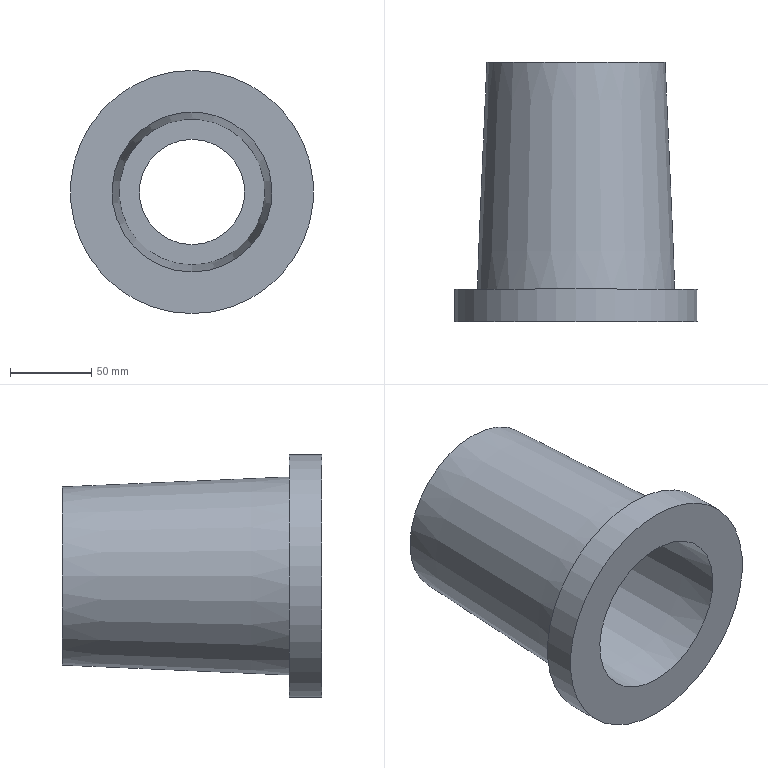Component | NX | BASE | 1 solid | 17 faces | box 150 x 160 x 150 mm | volume 897725 mm3 | cylinder 6 | cone 6 | plane 5 | commonest cylinder face diameters 82 x2 8.5 x2 150 x1 65 x1
STEP:
#1=CARTESIAN_POINT('',(0.,0.,0.));
#2=DIRECTION('',(0.,0.,1.));
#3=DIRECTION('',(1.,0.,0.));
#4=AXIS2_PLACEMENT_3D('',#1,#2,#3);
#5=CARTESIAN_POINT('',(-4.244,159.25,-40.78));
#6=VERTEX_POINT('',#5);
#7=CARTESIAN_POINT('',(-4.991,160.,-40.695));
#8=VERTEX_POINT('',#7);
#9=CARTESIAN_POINT('',(-4.244,159.25,-40.78));
#10=CARTESIAN_POINT('',(-4.493,159.5,-40.754));
#11=CARTESIAN_POINT('',(-4.742,159.75,-40.726));
#12=CARTESIAN_POINT('',(-4.991,160.,-40.695));
#13=B_SPLINE_CURVE_WITH_KNOTS('',3,(#9,#10,#11,#12),.UNSPECIFIED.,.F.,.F.,(4,4),(0.,1.),.PIECEWISE_BEZIER_KNOTS.);
#14=CARTESIAN_POINT('',(0.,0.,0.));
#15=DIRECTION('',(0.,-1.,0.));
#16=DIRECTION('',(0.,0.,-1.));
#17=AXIS2_PLACEMENT_3D('',#14,#15,#16);
#18=CYLINDRICAL_SURFACE('',#17,41.);
#19=CARTESIAN_POINT('',(6.179,-159.25));
#20=CARTESIAN_POINT('',(6.161,-160.));
#21=B_SPLINE_CURVE_WITH_KNOTS('',1,(#19,#20),.UNSPECIFIED.,.F.,.F.,(2,2),(0.,1.),.PIECEWISE_BEZIER_KNOTS.);
#22=(GEOMETRIC_REPRESENTATION_CONTEXT(2)PARAMETRIC_REPRESENTATION_CONTEXT()REPRESENTATION_CONTEXT('',''));
#23=DEFINITIONAL_REPRESENTATION('',(#21),#22);
#24=PCURVE('',#18,#23);
#25=CARTESIAN_POINT('',(0.,160.,-41.));
#26=DIRECTION('',(0.,1.,0.));
#27=DIRECTION('',(0.,0.,1.));
#28=AXIS2_PLACEMENT_3D('',#25,#26,#27);
#29=CONICAL_SURFACE('',#28,5.,0.7854);
#30=CARTESIAN_POINT('',(4.764,-0.75));
#31=CARTESIAN_POINT('',(4.773,0.));
#32=B_SPLINE_CURVE_WITH_KNOTS('',1,(#30,#31),.UNSPECIFIED.,.F.,.F.,(2,2),(0.,1.),.PIECEWISE_BEZIER_KNOTS.);
#33=(GEOMETRIC_REPRESENTATION_CONTEXT(2)PARAMETRIC_REPRESENTATION_CONTEXT()REPRESENTATION_CONTEXT('',''));
#34=DEFINITIONAL_REPRESENTATION('',(#32),#33);
#35=PCURVE('',#29,#34);
#36=SURFACE_CURVE('',#13,(#24,#35),.PCURVE_S1.);
#37=EDGE_CURVE('',#6,#8,#36,.T.);
#38=ORIENTED_EDGE('',*,*,#37,.F.);
#39=CARTESIAN_POINT('',(-4.244,140.,-40.78));
#40=VERTEX_POINT('',#39);
#41=CARTESIAN_POINT('',(-4.244,150.,-40.78));
#42=DIRECTION('',(0.,1.,0.));
#43=VECTOR('',#42,1.);
#44=LINE('',#41,#43);
#45=CARTESIAN_POINT('',(6.179,-150.));
#46=DIRECTION('',(0.,-1.));
#47=VECTOR('',#46,1.);
#48=LINE('',#45,#47);
#49=(GEOMETRIC_REPRESENTATION_CONTEXT(2)PARAMETRIC_REPRESENTATION_CONTEXT()REPRESENTATION_CONTEXT('',''));
#50=DEFINITIONAL_REPRESENTATION('',(#48),#49);
#51=PCURVE('',#18,#50);
#52=CARTESIAN_POINT('',(0.,160.,-41.));
#53=DIRECTION('',(0.,-1.,0.));
#54=DIRECTION('',(0.,0.,-1.));
#55=AXIS2_PLACEMENT_3D('',#52,#53,#54);
#56=CYLINDRICAL_SURFACE('',#55,4.25);
#57=CARTESIAN_POINT('',(-1.623,10.));
#58=DIRECTION('',(0.,-1.));
#59=VECTOR('',#58,1.);
#60=LINE('',#57,#59);
#61=(GEOMETRIC_REPRESENTATION_CONTEXT(2)PARAMETRIC_REPRESENTATION_CONTEXT()REPRESENTATION_CONTEXT('',''));
#62=DEFINITIONAL_REPRESENTATION('',(#60),#61);
#63=PCURVE('',#56,#62);
#64=SURFACE_CURVE('',#44,(#51,#63),.PCURVE_S1.);
#65=EDGE_CURVE('',#40,#6,#64,.T.);
#66=ORIENTED_EDGE('',*,*,#65,.F.);
#67=CARTESIAN_POINT('',(-4.244,140.,40.78));
#68=VERTEX_POINT('',#67);
#69=CARTESIAN_POINT('',(0.,140.,0.));
#70=DIRECTION('',(0.,-1.,0.));
#71=DIRECTION('',(0.,0.,-1.));
#72=AXIS2_PLACEMENT_3D('',#69,#70,#71);
#73=CIRCLE('',#72,41.);
#74=CARTESIAN_POINT('',(-0.,-140.));
#75=DIRECTION('',(1.,0.));
#76=VECTOR('',#75,1.);
#77=LINE('',#74,#76);
#78=(GEOMETRIC_REPRESENTATION_CONTEXT(2)PARAMETRIC_REPRESENTATION_CONTEXT()REPRESENTATION_CONTEXT('',''));
#79=DEFINITIONAL_REPRESENTATION('',(#77),#78);
#80=PCURVE('',#18,#79);
#81=CARTESIAN_POINT('',(-32.5,140.,0.));
#82=DIRECTION('',(0.,-1.,0.));
#83=DIRECTION('',(0.,0.,-1.));
#84=AXIS2_PLACEMENT_3D('',#81,#82,#83);
#85=PLANE('',#84);
#86=CARTESIAN_POINT('',(0.,32.5));
#87=DIRECTION('',(1.,0.));
#88=AXIS2_PLACEMENT_2D('',#86,#87);
#89=CIRCLE('',#88,41.);
#90=(GEOMETRIC_REPRESENTATION_CONTEXT(2)PARAMETRIC_REPRESENTATION_CONTEXT()REPRESENTATION_CONTEXT('',''));
#91=DEFINITIONAL_REPRESENTATION('',(#89),#90);
#92=PCURVE('',#85,#91);
#93=SURFACE_CURVE('',#73,(#80,#92),.PCURVE_S1.);
#94=EDGE_CURVE('',#68,#40,#93,.T.);
#95=ORIENTED_EDGE('',*,*,#94,.F.);
#96=CARTESIAN_POINT('',(-4.244,159.25,40.78));
#97=VERTEX_POINT('',#96);
#98=CARTESIAN_POINT('',(-4.244,150.,40.78));
#99=DIRECTION('',(0.,-1.,0.));
#100=VECTOR('',#99,1.);
#101=LINE('',#98,#100);
#102=CARTESIAN_POINT('',(3.245,-150.));
#103=DIRECTION('',(0.,1.));
#104=VECTOR('',#103,1.);
#105=LINE('',#102,#104);
#106=(GEOMETRIC_REPRESENTATION_CONTEXT(2)PARAMETRIC_REPRESENTATION_CONTEXT()REPRESENTATION_CONTEXT('',''));
#107=DEFINITIONAL_REPRESENTATION('',(#105),#106);
#108=PCURVE('',#18,#107);
#109=CARTESIAN_POINT('',(0.,160.,41.));
#110=DIRECTION('',(0.,-1.,0.));
#111=DIRECTION('',(0.,0.,-1.));
#112=AXIS2_PLACEMENT_3D('',#109,#110,#111);
#113=CYLINDRICAL_SURFACE('',#112,4.25);
#114=CARTESIAN_POINT('',(4.764,10.));
#115=DIRECTION('',(0.,1.));
#116=VECTOR('',#115,1.);
#117=LINE('',#114,#116);
#118=(GEOMETRIC_REPRESENTATION_CONTEXT(2)PARAMETRIC_REPRESENTATION_CONTEXT()REPRESENTATION_CONTEXT('',''));
#119=DEFINITIONAL_REPRESENTATION('',(#117),#118);
#120=PCURVE('',#113,#119);
#121=SURFACE_CURVE('',#101,(#108,#120),.PCURVE_S1.);
#122=EDGE_CURVE('',#97,#68,#121,.T.);
#123=ORIENTED_EDGE('',*,*,#122,.F.);
#124=CARTESIAN_POINT('',(-4.991,160.,40.695));
#125=VERTEX_POINT('',#124);
#126=CARTESIAN_POINT('',(-4.991,160.,40.695));
#127=CARTESIAN_POINT('',(-4.742,159.75,40.726));
#128=CARTESIAN_POINT('',(-4.493,159.5,40.754));
#129=CARTESIAN_POINT('',(-4.244,159.25,40.78));
#130=B_SPLINE_CURVE_WITH_KNOTS('',3,(#126,#127,#128,#129),.UNSPECIFIED.,.F.,.F.,(4,4),(0.,1.),.PIECEWISE_BEZIER_KNOTS.);
#131=CARTESIAN_POINT('',(3.264,-160.));
#132=CARTESIAN_POINT('',(3.245,-159.25));
#133=B_SPLINE_CURVE_WITH_KNOTS('',1,(#131,#132),.UNSPECIFIED.,.F.,.F.,(2,2),(0.,1.),.PIECEWISE_BEZIER_KNOTS.);
#134=(GEOMETRIC_REPRESENTATION_CONTEXT(2)PARAMETRIC_REPRESENTATION_CONTEXT()REPRESENTATION_CONTEXT('',''));
#135=DEFINITIONAL_REPRESENTATION('',(#133),#134);
#136=PCURVE('',#18,#135);
#137=CARTESIAN_POINT('',(0.,160.,41.));
#138=DIRECTION('',(0.,1.,0.));
#139=DIRECTION('',(0.,0.,1.));
#140=AXIS2_PLACEMENT_3D('',#137,#138,#139);
#141=CONICAL_SURFACE('',#140,5.,0.7854);
#142=CARTESIAN_POINT('',(-1.632,0.));
#143=CARTESIAN_POINT('',(-1.623,-0.75));
#144=B_SPLINE_CURVE_WITH_KNOTS('',1,(#142,#143),.UNSPECIFIED.,.F.,.F.,(2,2),(0.,1.),.PIECEWISE_BEZIER_KNOTS.);
#145=(GEOMETRIC_REPRESENTATION_CONTEXT(2)PARAMETRIC_REPRESENTATION_CONTEXT()REPRESENTATION_CONTEXT('',''));
#146=DEFINITIONAL_REPRESENTATION('',(#144),#145);
#147=PCURVE('',#141,#146);
#148=SURFACE_CURVE('',#130,(#136,#147),.PCURVE_S1.);
#149=EDGE_CURVE('',#125,#97,#148,.T.);
#150=ORIENTED_EDGE('',*,*,#149,.F.);
#151=CARTESIAN_POINT('',(0.,160.,0.));
#152=DIRECTION('',(0.,-1.,0.));
#153=DIRECTION('',(0.,0.,-1.));
#154=AXIS2_PLACEMENT_3D('',#151,#152,#153);
#155=CIRCLE('',#154,41.);
#156=CARTESIAN_POINT('',(-0.,-160.));
#157=DIRECTION('',(1.,0.));
#158=VECTOR('',#157,1.);
#159=LINE('',#156,#158);
#160=(GEOMETRIC_REPRESENTATION_CONTEXT(2)PARAMETRIC_REPRESENTATION_CONTEXT()REPRESENTATION_CONTEXT('',''));
#161=DEFINITIONAL_REPRESENTATION('',(#159),#160);
#162=PCURVE('',#18,#161);
#163=CARTESIAN_POINT('',(-41.,160.,0.));
#164=DIRECTION('',(0.,-1.,0.));
#165=DIRECTION('',(0.,0.,-1.));
#166=AXIS2_PLACEMENT_3D('',#163,#164,#165);
#167=PLANE('',#166);
#168=CARTESIAN_POINT('',(0.,41.));
#169=DIRECTION('',(1.,0.));
#170=AXIS2_PLACEMENT_2D('',#168,#169);
#171=CIRCLE('',#170,41.);
#172=(GEOMETRIC_REPRESENTATION_CONTEXT(2)PARAMETRIC_REPRESENTATION_CONTEXT()REPRESENTATION_CONTEXT('',''));
#173=DEFINITIONAL_REPRESENTATION('',(#171),#172);
#174=PCURVE('',#167,#173);
#175=SURFACE_CURVE('',#155,(#162,#174),.PCURVE_S1.);
#176=EDGE_CURVE('',#125,#8,#175,.T.);
#177=ORIENTED_EDGE('',*,*,#176,.T.);
#178=EDGE_LOOP('',(#38,#66,#95,#123,#150,#177));
#179=FACE_BOUND('',#178,.F.);
#180=ADVANCED_FACE('',(#179),#18,.F.);
#181=CARTESIAN_POINT('',(0.,20.,-61.113));
#182=VERTEX_POINT('',#181);
#183=CARTESIAN_POINT('',(0.,20.,0.));
#184=DIRECTION('',(0.,-1.,0.));
#185=DIRECTION('',(0.,0.,-1.));
#186=AXIS2_PLACEMENT_3D('',#183,#184,#185);
#187=CIRCLE('',#186,61.113);
#188=CARTESIAN_POINT('',(0.,160.,0.));
#189=DIRECTION('',(0.,-1.,0.));
#190=DIRECTION('',(0.,0.,-1.));
#191=AXIS2_PLACEMENT_3D('',#188,#189,#190);
#192=CONICAL_SURFACE('',#191,55.,0.04363);
#193=CARTESIAN_POINT('',(0.,140.));
#194=DIRECTION('',(1.,0.));
#195=VECTOR('',#194,1.);
#196=LINE('',#193,#195);
#197=(GEOMETRIC_REPRESENTATION_CONTEXT(2)PARAMETRIC_REPRESENTATION_CONTEXT()REPRESENTATION_CONTEXT('',''));
#198=DEFINITIONAL_REPRESENTATION('',(#196),#197);
#199=PCURVE('',#192,#198);
#200=CARTESIAN_POINT('',(-61.113,20.,0.));
#201=DIRECTION('',(0.,-1.,0.));
#202=DIRECTION('',(0.,0.,-1.));
#203=AXIS2_PLACEMENT_3D('',#200,#201,#202);
#204=PLANE('',#203);
#205=CARTESIAN_POINT('',(0.,61.113));
#206=DIRECTION('',(1.,0.));
#207=AXIS2_PLACEMENT_2D('',#205,#206);
#208=CIRCLE('',#207,61.113);
#209=(GEOMETRIC_REPRESENTATION_CONTEXT(2)PARAMETRIC_REPRESENTATION_CONTEXT()REPRESENTATION_CONTEXT('',''));
#210=DEFINITIONAL_REPRESENTATION('',(#208),#209);
#211=PCURVE('',#204,#210);
#212=SURFACE_CURVE('',#187,(#199,#211),.PCURVE_S1.);
#213=EDGE_CURVE('',#182,#182,#212,.T.);
#214=ORIENTED_EDGE('',*,*,#213,.F.);
#215=CARTESIAN_POINT('',(0.,160.,-55.));
#216=VERTEX_POINT('',#215);
#217=CARTESIAN_POINT('',(-0.,160.,-55.));
#218=CARTESIAN_POINT('',(-0.,20.,-61.113));
#219=B_SPLINE_CURVE_WITH_KNOTS('',1,(#217,#218),.UNSPECIFIED.,.F.,.F.,(2,2),(0.,140.133),.PIECEWISE_BEZIER_KNOTS.);
#220=CARTESIAN_POINT('',(0.,0.));
#221=DIRECTION('',(0.,1.));
#222=VECTOR('',#221,1.);
#223=LINE('',#220,#222);
#224=(GEOMETRIC_REPRESENTATION_CONTEXT(2)PARAMETRIC_REPRESENTATION_CONTEXT()REPRESENTATION_CONTEXT('',''));
#225=DEFINITIONAL_REPRESENTATION('',(#223),#224);
#226=PCURVE('',#192,#225);
#227=CARTESIAN_POINT('',(6.283,0.));
#228=DIRECTION('',(0.,1.));
#229=VECTOR('',#228,1.);
#230=LINE('',#227,#229);
#231=(GEOMETRIC_REPRESENTATION_CONTEXT(2)PARAMETRIC_REPRESENTATION_CONTEXT()REPRESENTATION_CONTEXT('',''));
#232=DEFINITIONAL_REPRESENTATION('',(#230),#231);
#233=PCURVE('',#192,#232);
#234=SEAM_CURVE('',#219,(#226,#233),.PCURVE_S1.);
#235=EDGE_CURVE('',#216,#182,#234,.T.);
#236=ORIENTED_EDGE('',*,*,#235,.F.);
#237=CARTESIAN_POINT('',(0.,160.,0.));
#238=DIRECTION('',(0.,-1.,0.));
#239=DIRECTION('',(0.,0.,-1.));
#240=AXIS2_PLACEMENT_3D('',#237,#238,#239);
#241=CIRCLE('',#240,55.);
#242=CARTESIAN_POINT('',(0.,0.));
#243=DIRECTION('',(1.,0.));
#244=VECTOR('',#243,1.);
#245=LINE('',#242,#244);
#246=(GEOMETRIC_REPRESENTATION_CONTEXT(2)PARAMETRIC_REPRESENTATION_CONTEXT()REPRESENTATION_CONTEXT('',''));
#247=DEFINITIONAL_REPRESENTATION('',(#245),#246);
#248=PCURVE('',#192,#247);
#249=CARTESIAN_POINT('',(0.,41.));
#250=DIRECTION('',(1.,0.));
#251=AXIS2_PLACEMENT_2D('',#249,#250);
#252=CIRCLE('',#251,55.);
#253=(GEOMETRIC_REPRESENTATION_CONTEXT(2)PARAMETRIC_REPRESENTATION_CONTEXT()REPRESENTATION_CONTEXT('',''));
#254=DEFINITIONAL_REPRESENTATION('',(#252),#253);
#255=PCURVE('',#167,#254);
#256=SURFACE_CURVE('',#241,(#248,#255),.PCURVE_S1.);
#257=EDGE_CURVE('',#216,#216,#256,.T.);
#258=ORIENTED_EDGE('',*,*,#257,.T.);
#259=ORIENTED_EDGE('',*,*,#235,.T.);
#260=EDGE_LOOP('',(#214,#236,#258,#259));
#261=FACE_BOUND('',#260,.T.);
#262=ADVANCED_FACE('',(#261),#192,.T.);
#263=CARTESIAN_POINT('',(0.,20.,-75.));
#264=VERTEX_POINT('',#263);
#265=CARTESIAN_POINT('',(0.,20.,0.));
#266=DIRECTION('',(0.,-1.,0.));
#267=DIRECTION('',(0.,0.,-1.));
#268=AXIS2_PLACEMENT_3D('',#265,#266,#267);
#269=CIRCLE('',#268,75.);
#270=CARTESIAN_POINT('',(0.,61.113));
#271=DIRECTION('',(1.,0.));
#272=AXIS2_PLACEMENT_2D('',#270,#271);
#273=CIRCLE('',#272,75.);
#274=(GEOMETRIC_REPRESENTATION_CONTEXT(2)PARAMETRIC_REPRESENTATION_CONTEXT()REPRESENTATION_CONTEXT('',''));
#275=DEFINITIONAL_REPRESENTATION('',(#273),#274);
#276=PCURVE('',#204,#275);
#277=CARTESIAN_POINT('',(0.,0.,0.));
#278=DIRECTION('',(0.,-1.,0.));
#279=DIRECTION('',(0.,0.,-1.));
#280=AXIS2_PLACEMENT_3D('',#277,#278,#279);
#281=CYLINDRICAL_SURFACE('',#280,75.);
#282=CARTESIAN_POINT('',(0.,-20.));
#283=DIRECTION('',(1.,0.));
#284=VECTOR('',#283,1.);
#285=LINE('',#282,#284);
#286=(GEOMETRIC_REPRESENTATION_CONTEXT(2)PARAMETRIC_REPRESENTATION_CONTEXT()REPRESENTATION_CONTEXT('',''));
#287=DEFINITIONAL_REPRESENTATION('',(#285),#286);
#288=PCURVE('',#281,#287);
#289=SURFACE_CURVE('',#269,(#276,#288),.PCURVE_S1.);
#290=EDGE_CURVE('',#264,#264,#289,.T.);
#291=ORIENTED_EDGE('',*,*,#290,.F.);
#292=EDGE_LOOP('',(#291));
#293=FACE_BOUND('',#292,.T.);
#294=ORIENTED_EDGE('',*,*,#213,.T.);
#295=EDGE_LOOP('',(#294));
#296=FACE_BOUND('',#295,.T.);
#297=ADVANCED_FACE('',(#293,#296),#204,.F.);
#298=CARTESIAN_POINT('',(0.,-0.,-75.));
#299=VERTEX_POINT('',#298);
#300=CARTESIAN_POINT('',(0.,-0.,0.));
#301=DIRECTION('',(0.,-1.,0.));
#302=DIRECTION('',(0.,0.,-1.));
#303=AXIS2_PLACEMENT_3D('',#300,#301,#302);
#304=CIRCLE('',#303,75.);
#305=CARTESIAN_POINT('',(0.,0.));
#306=DIRECTION('',(1.,0.));
#307=VECTOR('',#306,1.);
#308=LINE('',#305,#307);
#309=(GEOMETRIC_REPRESENTATION_CONTEXT(2)PARAMETRIC_REPRESENTATION_CONTEXT()REPRESENTATION_CONTEXT('',''));
#310=DEFINITIONAL_REPRESENTATION('',(#308),#309);
#311=PCURVE('',#281,#310);
#312=CARTESIAN_POINT('',(-75.,-0.,0.));
#313=DIRECTION('',(0.,1.,0.));
#314=DIRECTION('',(0.,0.,1.));
#315=AXIS2_PLACEMENT_3D('',#312,#313,#314);
#316=PLANE('',#315);
#317=CARTESIAN_POINT('',(-75.,75.));
#318=CARTESIAN_POINT('',(-75.,204.904));
#319=CARTESIAN_POINT('',(37.5,139.952));
#320=CARTESIAN_POINT('',(150.,75.));
#321=CARTESIAN_POINT('',(37.5,10.048));
#322=CARTESIAN_POINT('',(-75.,-54.904));
#323=CARTESIAN_POINT('',(-75.,75.));
#324=(BOUNDED_CURVE()B_SPLINE_CURVE(2,(#317,#318,#319,#320,#321,#322,#323),.UNSPECIFIED.,.T.,.F.)B_SPLINE_CURVE_WITH_KNOTS((1,2,2,2,2,1),(-2.094,0.,2.094,4.189,6.283,8.378),.UNSPECIFIED.)CURVE()GEOMETRIC_REPRESENTATION_ITEM()RATIONAL_B_SPLINE_CURVE((1.,0.5,1.,0.5,1.,0.5,1.))REPRESENTATION_ITEM(''));
#325=(GEOMETRIC_REPRESENTATION_CONTEXT(2)PARAMETRIC_REPRESENTATION_CONTEXT()REPRESENTATION_CONTEXT('',''));
#326=DEFINITIONAL_REPRESENTATION('',(#324),#325);
#327=PCURVE('',#316,#326);
#328=SURFACE_CURVE('',#304,(#311,#327),.PCURVE_S1.);
#329=EDGE_CURVE('',#299,#299,#328,.T.);
#330=ORIENTED_EDGE('',*,*,#329,.F.);
#331=CARTESIAN_POINT('',(-0.,20.,-75.));
#332=CARTESIAN_POINT('',(-0.,-0.,-75.));
#333=B_SPLINE_CURVE_WITH_KNOTS('',1,(#331,#332),.UNSPECIFIED.,.F.,.F.,(2,2),(-20.,0.),.PIECEWISE_BEZIER_KNOTS.);
#334=CARTESIAN_POINT('',(0.,0.));
#335=DIRECTION('',(0.,1.));
#336=VECTOR('',#335,1.);
#337=LINE('',#334,#336);
#338=(GEOMETRIC_REPRESENTATION_CONTEXT(2)PARAMETRIC_REPRESENTATION_CONTEXT()REPRESENTATION_CONTEXT('',''));
#339=DEFINITIONAL_REPRESENTATION('',(#337),#338);
#340=PCURVE('',#281,#339);
#341=CARTESIAN_POINT('',(6.283,0.));
#342=DIRECTION('',(0.,1.));
#343=VECTOR('',#342,1.);
#344=LINE('',#341,#343);
#345=(GEOMETRIC_REPRESENTATION_CONTEXT(2)PARAMETRIC_REPRESENTATION_CONTEXT()REPRESENTATION_CONTEXT('',''));
#346=DEFINITIONAL_REPRESENTATION('',(#344),#345);
#347=PCURVE('',#281,#346);
#348=SEAM_CURVE('',#333,(#340,#347),.PCURVE_S1.);
#349=EDGE_CURVE('',#264,#299,#348,.T.);
#350=ORIENTED_EDGE('',*,*,#349,.F.);
#351=ORIENTED_EDGE('',*,*,#290,.T.);
#352=ORIENTED_EDGE('',*,*,#349,.T.);
#353=EDGE_LOOP('',(#330,#350,#351,#352));
#354=FACE_BOUND('',#353,.T.);
#355=ADVANCED_FACE('',(#354),#281,.T.);
#356=CARTESIAN_POINT('',(0.,-0.,-49.366));
#357=VERTEX_POINT('',#356);
#358=CARTESIAN_POINT('',(0.,-0.,0.));
#359=DIRECTION('',(0.,-1.,0.));
#360=DIRECTION('',(0.,0.,-1.));
#361=AXIS2_PLACEMENT_3D('',#358,#359,#360);
#362=CIRCLE('',#361,49.366);
#363=CARTESIAN_POINT('',(-49.366,75.));
#364=CARTESIAN_POINT('',(-49.366,160.505));
#365=CARTESIAN_POINT('',(24.683,117.752));
#366=CARTESIAN_POINT('',(98.732,75.));
#367=CARTESIAN_POINT('',(24.683,32.248));
#368=CARTESIAN_POINT('',(-49.366,-10.505));
#369=CARTESIAN_POINT('',(-49.366,75.));
#370=(BOUNDED_CURVE()B_SPLINE_CURVE(2,(#363,#364,#365,#366,#367,#368,#369),.UNSPECIFIED.,.T.,.F.)B_SPLINE_CURVE_WITH_KNOTS((1,2,2,2,2,1),(-2.094,0.,2.094,4.189,6.283,8.378),.UNSPECIFIED.)CURVE()GEOMETRIC_REPRESENTATION_ITEM()RATIONAL_B_SPLINE_CURVE((1.,0.5,1.,0.5,1.,0.5,1.))REPRESENTATION_ITEM(''));
#371=(GEOMETRIC_REPRESENTATION_CONTEXT(2)PARAMETRIC_REPRESENTATION_CONTEXT()REPRESENTATION_CONTEXT('',''));
#372=DEFINITIONAL_REPRESENTATION('',(#370),#371);
#373=PCURVE('',#316,#372);
#374=CARTESIAN_POINT('',(0.,-0.,0.));
#375=DIRECTION('',(0.,-1.,0.));
#376=DIRECTION('',(0.,0.,-1.));
#377=AXIS2_PLACEMENT_3D('',#374,#375,#376);
#378=CONICAL_SURFACE('',#377,49.366,0.04363);
#379=CARTESIAN_POINT('',(0.,0.));
#380=DIRECTION('',(1.,0.));
#381=VECTOR('',#380,1.);
#382=LINE('',#379,#381);
#383=(GEOMETRIC_REPRESENTATION_CONTEXT(2)PARAMETRIC_REPRESENTATION_CONTEXT()REPRESENTATION_CONTEXT('',''));
#384=DEFINITIONAL_REPRESENTATION('',(#382),#383);
#385=PCURVE('',#378,#384);
#386=SURFACE_CURVE('',#362,(#373,#385),.PCURVE_S1.);
#387=EDGE_CURVE('',#357,#357,#386,.T.);
#388=ORIENTED_EDGE('',*,*,#387,.F.);
#389=EDGE_LOOP('',(#388));
#390=FACE_BOUND('',#389,.T.);
#391=ORIENTED_EDGE('',*,*,#329,.T.);
#392=EDGE_LOOP('',(#391));
#393=FACE_BOUND('',#392,.T.);
#394=ADVANCED_FACE('',(#390,#393),#316,.F.);
#395=CARTESIAN_POINT('',(0.,100.,-45.));
#396=VERTEX_POINT('',#395);
#397=CARTESIAN_POINT('',(0.,100.,0.));
#398=DIRECTION('',(0.,-1.,0.));
#399=DIRECTION('',(0.,0.,-1.));
#400=AXIS2_PLACEMENT_3D('',#397,#398,#399);
#401=CIRCLE('',#400,45.);
#402=CARTESIAN_POINT('',(0.,-100.));
#403=DIRECTION('',(1.,0.));
#404=VECTOR('',#403,1.);
#405=LINE('',#402,#404);
#406=(GEOMETRIC_REPRESENTATION_CONTEXT(2)PARAMETRIC_REPRESENTATION_CONTEXT()REPRESENTATION_CONTEXT('',''));
#407=DEFINITIONAL_REPRESENTATION('',(#405),#406);
#408=PCURVE('',#378,#407);
#409=CARTESIAN_POINT('',(-45.,100.,0.));
#410=DIRECTION('',(0.,1.,0.));
#411=DIRECTION('',(0.,0.,1.));
#412=AXIS2_PLACEMENT_3D('',#409,#410,#411);
#413=PLANE('',#412);
#414=CARTESIAN_POINT('',(-45.,45.));
#415=CARTESIAN_POINT('',(-45.,122.942));
#416=CARTESIAN_POINT('',(22.5,83.971));
#417=CARTESIAN_POINT('',(90.,45.));
#418=CARTESIAN_POINT('',(22.5,6.029));
#419=CARTESIAN_POINT('',(-45.,-32.942));
#420=CARTESIAN_POINT('',(-45.,45.));
#421=(BOUNDED_CURVE()B_SPLINE_CURVE(2,(#414,#415,#416,#417,#418,#419,#420),.UNSPECIFIED.,.T.,.F.)B_SPLINE_CURVE_WITH_KNOTS((1,2,2,2,2,1),(-2.094,0.,2.094,4.189,6.283,8.378),.UNSPECIFIED.)CURVE()GEOMETRIC_REPRESENTATION_ITEM()RATIONAL_B_SPLINE_CURVE((1.,0.5,1.,0.5,1.,0.5,1.))REPRESENTATION_ITEM(''));
#422=(GEOMETRIC_REPRESENTATION_CONTEXT(2)PARAMETRIC_REPRESENTATION_CONTEXT()REPRESENTATION_CONTEXT('',''));
#423=DEFINITIONAL_REPRESENTATION('',(#421),#422);
#424=PCURVE('',#413,#423);
#425=SURFACE_CURVE('',#401,(#408,#424),.PCURVE_S1.);
#426=EDGE_CURVE('',#396,#396,#425,.T.);
#427=ORIENTED_EDGE('',*,*,#426,.T.);
#428=CARTESIAN_POINT('',(0.,100.,-45.));
#429=CARTESIAN_POINT('',(0.,-0.,-49.366));
#430=B_SPLINE_CURVE_WITH_KNOTS('',1,(#428,#429),.UNSPECIFIED.,.F.,.F.,(2,2),(-100.095,0.),.PIECEWISE_BEZIER_KNOTS.);
#431=CARTESIAN_POINT('',(6.283,0.));
#432=DIRECTION('',(0.,1.));
#433=VECTOR('',#432,1.);
#434=LINE('',#431,#433);
#435=(GEOMETRIC_REPRESENTATION_CONTEXT(2)PARAMETRIC_REPRESENTATION_CONTEXT()REPRESENTATION_CONTEXT('',''));
#436=DEFINITIONAL_REPRESENTATION('',(#434),#435);
#437=PCURVE('',#378,#436);
#438=CARTESIAN_POINT('',(0.,0.));
#439=DIRECTION('',(0.,1.));
#440=VECTOR('',#439,1.);
#441=LINE('',#438,#440);
#442=(GEOMETRIC_REPRESENTATION_CONTEXT(2)PARAMETRIC_REPRESENTATION_CONTEXT()REPRESENTATION_CONTEXT('',''));
#443=DEFINITIONAL_REPRESENTATION('',(#441),#442);
#444=PCURVE('',#378,#443);
#445=SEAM_CURVE('',#430,(#437,#444),.PCURVE_S1.);
#446=EDGE_CURVE('',#396,#357,#445,.T.);
#447=ORIENTED_EDGE('',*,*,#446,.T.);
#448=ORIENTED_EDGE('',*,*,#387,.F.);
#449=ORIENTED_EDGE('',*,*,#446,.F.);
#450=EDGE_LOOP('',(#427,#447,#448,#449));
#451=FACE_BOUND('',#450,.F.);
#452=ADVANCED_FACE('',(#451),#378,.F.);
#453=CARTESIAN_POINT('',(0.,100.,-32.5));
#454=VERTEX_POINT('',#453);
#455=CARTESIAN_POINT('',(0.,100.,0.));
#456=DIRECTION('',(0.,-1.,0.));
#457=DIRECTION('',(0.,0.,-1.));
#458=AXIS2_PLACEMENT_3D('',#455,#456,#457);
#459=CIRCLE('',#458,32.5);
#460=CARTESIAN_POINT('',(-32.5,45.));
#461=CARTESIAN_POINT('',(-32.5,101.292));
#462=CARTESIAN_POINT('',(16.25,73.146));
#463=CARTESIAN_POINT('',(65.,45.));
#464=CARTESIAN_POINT('',(16.25,16.854));
#465=CARTESIAN_POINT('',(-32.5,-11.292));
#466=CARTESIAN_POINT('',(-32.5,45.));
#467=(BOUNDED_CURVE()B_SPLINE_CURVE(2,(#460,#461,#462,#463,#464,#465,#466),.UNSPECIFIED.,.T.,.F.)B_SPLINE_CURVE_WITH_KNOTS((1,2,2,2,2,1),(-2.094,0.,2.094,4.189,6.283,8.378),.UNSPECIFIED.)CURVE()GEOMETRIC_REPRESENTATION_ITEM()RATIONAL_B_SPLINE_CURVE((1.,0.5,1.,0.5,1.,0.5,1.))REPRESENTATION_ITEM(''));
#468=(GEOMETRIC_REPRESENTATION_CONTEXT(2)PARAMETRIC_REPRESENTATION_CONTEXT()REPRESENTATION_CONTEXT('',''));
#469=DEFINITIONAL_REPRESENTATION('',(#467),#468);
#470=PCURVE('',#413,#469);
#471=CARTESIAN_POINT('',(0.,0.,0.));
#472=DIRECTION('',(0.,-1.,0.));
#473=DIRECTION('',(0.,0.,-1.));
#474=AXIS2_PLACEMENT_3D('',#471,#472,#473);
#475=CYLINDRICAL_SURFACE('',#474,32.5);
#476=CARTESIAN_POINT('',(0.,-100.));
#477=DIRECTION('',(1.,0.));
#478=VECTOR('',#477,1.);
#479=LINE('',#476,#478);
#480=(GEOMETRIC_REPRESENTATION_CONTEXT(2)PARAMETRIC_REPRESENTATION_CONTEXT()REPRESENTATION_CONTEXT('',''));
#481=DEFINITIONAL_REPRESENTATION('',(#479),#480);
#482=PCURVE('',#475,#481);
#483=SURFACE_CURVE('',#459,(#470,#482),.PCURVE_S1.);
#484=EDGE_CURVE('',#454,#454,#483,.T.);
#485=ORIENTED_EDGE('',*,*,#484,.F.);
#486=EDGE_LOOP('',(#485));
#487=FACE_BOUND('',#486,.T.);
#488=ORIENTED_EDGE('',*,*,#426,.T.);
#489=EDGE_LOOP('',(#488));
#490=FACE_BOUND('',#489,.T.);
#491=ADVANCED_FACE('',(#487,#490),#413,.F.);
#492=CARTESIAN_POINT('',(0.,140.,-32.5));
#493=VERTEX_POINT('',#492);
#494=CARTESIAN_POINT('',(0.,140.,0.));
#495=DIRECTION('',(0.,-1.,0.));
#496=DIRECTION('',(0.,0.,-1.));
#497=AXIS2_PLACEMENT_3D('',#494,#495,#496);
#498=CIRCLE('',#497,32.5);
#499=CARTESIAN_POINT('',(0.,-140.));
#500=DIRECTION('',(1.,0.));
#501=VECTOR('',#500,1.);
#502=LINE('',#499,#501);
#503=(GEOMETRIC_REPRESENTATION_CONTEXT(2)PARAMETRIC_REPRESENTATION_CONTEXT()REPRESENTATION_CONTEXT('',''));
#504=DEFINITIONAL_REPRESENTATION('',(#502),#503);
#505=PCURVE('',#475,#504);
#506=CARTESIAN_POINT('',(0.,32.5));
#507=DIRECTION('',(1.,0.));
#508=AXIS2_PLACEMENT_2D('',#506,#507);
#509=CIRCLE('',#508,32.5);
#510=(GEOMETRIC_REPRESENTATION_CONTEXT(2)PARAMETRIC_REPRESENTATION_CONTEXT()REPRESENTATION_CONTEXT('',''));
#511=DEFINITIONAL_REPRESENTATION('',(#509),#510);
#512=PCURVE('',#85,#511);
#513=SURFACE_CURVE('',#498,(#505,#512),.PCURVE_S1.);
#514=EDGE_CURVE('',#493,#493,#513,.T.);
#515=ORIENTED_EDGE('',*,*,#514,.T.);
#516=CARTESIAN_POINT('',(0.,140.,-32.5));
#517=CARTESIAN_POINT('',(0.,100.,-32.5));
#518=B_SPLINE_CURVE_WITH_KNOTS('',1,(#516,#517),.UNSPECIFIED.,.F.,.F.,(2,2),(-140.,-100.),.PIECEWISE_BEZIER_KNOTS.);
#519=CARTESIAN_POINT('',(6.283,0.));
#520=DIRECTION('',(0.,1.));
#521=VECTOR('',#520,1.);
#522=LINE('',#519,#521);
#523=(GEOMETRIC_REPRESENTATION_CONTEXT(2)PARAMETRIC_REPRESENTATION_CONTEXT()REPRESENTATION_CONTEXT('',''));
#524=DEFINITIONAL_REPRESENTATION('',(#522),#523);
#525=PCURVE('',#475,#524);
#526=CARTESIAN_POINT('',(0.,0.));
#527=DIRECTION('',(0.,1.));
#528=VECTOR('',#527,1.);
#529=LINE('',#526,#528);
#530=(GEOMETRIC_REPRESENTATION_CONTEXT(2)PARAMETRIC_REPRESENTATION_CONTEXT()REPRESENTATION_CONTEXT('',''));
#531=DEFINITIONAL_REPRESENTATION('',(#529),#530);
#532=PCURVE('',#475,#531);
#533=SEAM_CURVE('',#518,(#525,#532),.PCURVE_S1.);
#534=EDGE_CURVE('',#493,#454,#533,.T.);
#535=ORIENTED_EDGE('',*,*,#534,.T.);
#536=ORIENTED_EDGE('',*,*,#484,.F.);
#537=ORIENTED_EDGE('',*,*,#534,.F.);
#538=EDGE_LOOP('',(#515,#535,#536,#537));
#539=FACE_BOUND('',#538,.F.);
#540=ADVANCED_FACE('',(#539),#475,.F.);
#541=ORIENTED_EDGE('',*,*,#94,.F.);
#542=CARTESIAN_POINT('',(4.244,140.,40.78));
#543=VERTEX_POINT('',#542);
#544=CARTESIAN_POINT('',(0.,140.,41.));
#545=DIRECTION('',(0.,-1.,0.));
#546=DIRECTION('',(0.,0.,-1.));
#547=AXIS2_PLACEMENT_3D('',#544,#545,#546);
#548=CIRCLE('',#547,4.25);
#549=CARTESIAN_POINT('',(-41.,32.5));
#550=DIRECTION('',(1.,0.));
#551=AXIS2_PLACEMENT_2D('',#549,#550);
#552=CIRCLE('',#551,4.25);
#553=(GEOMETRIC_REPRESENTATION_CONTEXT(2)PARAMETRIC_REPRESENTATION_CONTEXT()REPRESENTATION_CONTEXT('',''));
#554=DEFINITIONAL_REPRESENTATION('',(#552),#553);
#555=PCURVE('',#85,#554);
#556=CARTESIAN_POINT('',(0.,140.,41.));
#557=DIRECTION('',(0.,1.,0.));
#558=DIRECTION('',(0.,0.,1.));
#559=AXIS2_PLACEMENT_3D('',#556,#557,#558);
#560=CONICAL_SURFACE('',#559,4.25,1.03);
#561=CARTESIAN_POINT('',(9.425,0.));
#562=DIRECTION('',(-1.,0.));
#563=VECTOR('',#562,1.);
#564=LINE('',#561,#563);
#565=(GEOMETRIC_REPRESENTATION_CONTEXT(2)PARAMETRIC_REPRESENTATION_CONTEXT()REPRESENTATION_CONTEXT('',''));
#566=DEFINITIONAL_REPRESENTATION('',(#564),#565);
#567=PCURVE('',#560,#566);
#568=SURFACE_CURVE('',#548,(#555,#567),.PCURVE_S1.);
#569=EDGE_CURVE('',#68,#543,#568,.T.);
#570=ORIENTED_EDGE('',*,*,#569,.T.);
#571=CARTESIAN_POINT('',(4.244,140.,-40.78));
#572=VERTEX_POINT('',#571);
#573=CARTESIAN_POINT('',(0.,140.,0.));
#574=DIRECTION('',(0.,-1.,0.));
#575=DIRECTION('',(0.,0.,-1.));
#576=AXIS2_PLACEMENT_3D('',#573,#574,#575);
#577=CIRCLE('',#576,41.);
#578=CARTESIAN_POINT('',(0.,32.5));
#579=DIRECTION('',(1.,0.));
#580=AXIS2_PLACEMENT_2D('',#578,#579);
#581=CIRCLE('',#580,41.);
#582=(GEOMETRIC_REPRESENTATION_CONTEXT(2)PARAMETRIC_REPRESENTATION_CONTEXT()REPRESENTATION_CONTEXT('',''));
#583=DEFINITIONAL_REPRESENTATION('',(#581),#582);
#584=PCURVE('',#85,#583);
#585=CARTESIAN_POINT('',(0.,0.,0.));
#586=DIRECTION('',(0.,-1.,0.));
#587=DIRECTION('',(0.,0.,-1.));
#588=AXIS2_PLACEMENT_3D('',#585,#586,#587);
#589=CYLINDRICAL_SURFACE('',#588,41.);
#590=CARTESIAN_POINT('',(0.,-140.));
#591=DIRECTION('',(1.,0.));
#592=VECTOR('',#591,1.);
#593=LINE('',#590,#592);
#594=(GEOMETRIC_REPRESENTATION_CONTEXT(2)PARAMETRIC_REPRESENTATION_CONTEXT()REPRESENTATION_CONTEXT('',''));
#595=DEFINITIONAL_REPRESENTATION('',(#593),#594);
#596=PCURVE('',#589,#595);
#597=SURFACE_CURVE('',#577,(#584,#596),.PCURVE_S1.);
#598=EDGE_CURVE('',#572,#543,#597,.T.);
#599=ORIENTED_EDGE('',*,*,#598,.F.);
#600=CARTESIAN_POINT('',(0.,140.,-36.75));
#601=VERTEX_POINT('',#600);
#602=CARTESIAN_POINT('',(0.,140.,-41.));
#603=DIRECTION('',(0.,-1.,0.));
#604=DIRECTION('',(0.,0.,-1.));
#605=AXIS2_PLACEMENT_3D('',#602,#603,#604);
#606=CIRCLE('',#605,4.25);
#607=CARTESIAN_POINT('',(41.,32.5));
#608=DIRECTION('',(1.,0.));
#609=AXIS2_PLACEMENT_2D('',#607,#608);
#610=CIRCLE('',#609,4.25);
#611=(GEOMETRIC_REPRESENTATION_CONTEXT(2)PARAMETRIC_REPRESENTATION_CONTEXT()REPRESENTATION_CONTEXT('',''));
#612=DEFINITIONAL_REPRESENTATION('',(#610),#611);
#613=PCURVE('',#85,#612);
#614=CARTESIAN_POINT('',(0.,140.,-41.));
#615=DIRECTION('',(0.,1.,0.));
#616=DIRECTION('',(0.,0.,1.));
#617=AXIS2_PLACEMENT_3D('',#614,#615,#616);
#618=CONICAL_SURFACE('',#617,4.25,1.03);
#619=CARTESIAN_POINT('',(3.142,0.));
#620=DIRECTION('',(-1.,0.));
#621=VECTOR('',#620,1.);
#622=LINE('',#619,#621);
#623=(GEOMETRIC_REPRESENTATION_CONTEXT(2)PARAMETRIC_REPRESENTATION_CONTEXT()REPRESENTATION_CONTEXT('',''));
#624=DEFINITIONAL_REPRESENTATION('',(#622),#623);
#625=PCURVE('',#618,#624);
#626=SURFACE_CURVE('',#606,(#613,#625),.PCURVE_S1.);
#627=EDGE_CURVE('',#572,#601,#626,.T.);
#628=ORIENTED_EDGE('',*,*,#627,.T.);
#629=CARTESIAN_POINT('',(0.,140.,-41.));
#630=DIRECTION('',(0.,-1.,0.));
#631=DIRECTION('',(0.,0.,-1.));
#632=AXIS2_PLACEMENT_3D('',#629,#630,#631);
#633=CIRCLE('',#632,4.25);
#634=CARTESIAN_POINT('',(41.,32.5));
#635=DIRECTION('',(1.,0.));
#636=AXIS2_PLACEMENT_2D('',#634,#635);
#637=CIRCLE('',#636,4.25);
#638=(GEOMETRIC_REPRESENTATION_CONTEXT(2)PARAMETRIC_REPRESENTATION_CONTEXT()REPRESENTATION_CONTEXT('',''));
#639=DEFINITIONAL_REPRESENTATION('',(#637),#638);
#640=PCURVE('',#85,#639);
#641=CARTESIAN_POINT('',(9.425,0.));
#642=DIRECTION('',(-1.,0.));
#643=VECTOR('',#642,1.);
#644=LINE('',#641,#643);
#645=(GEOMETRIC_REPRESENTATION_CONTEXT(2)PARAMETRIC_REPRESENTATION_CONTEXT()REPRESENTATION_CONTEXT('',''));
#646=DEFINITIONAL_REPRESENTATION('',(#644),#645);
#647=PCURVE('',#618,#646);
#648=SURFACE_CURVE('',#633,(#640,#647),.PCURVE_S1.);
#649=EDGE_CURVE('',#601,#40,#648,.T.);
#650=ORIENTED_EDGE('',*,*,#649,.T.);
#651=EDGE_LOOP('',(#541,#570,#599,#628,#650));
#652=FACE_BOUND('',#651,.T.);
#653=ORIENTED_EDGE('',*,*,#514,.T.);
#654=EDGE_LOOP('',(#653));
#655=FACE_BOUND('',#654,.T.);
#656=ADVANCED_FACE('',(#652,#655),#85,.F.);
#657=ORIENTED_EDGE('',*,*,#598,.F.);
#658=CARTESIAN_POINT('',(4.244,159.25,-40.78));
#659=VERTEX_POINT('',#658);
#660=CARTESIAN_POINT('',(4.244,150.,-40.78));
#661=DIRECTION('',(0.,-1.,0.));
#662=VECTOR('',#661,1.);
#663=LINE('',#660,#662);
#664=CARTESIAN_POINT('',(0.1037,-150.));
#665=DIRECTION('',(0.,1.));
#666=VECTOR('',#665,1.);
#667=LINE('',#664,#666);
#668=(GEOMETRIC_REPRESENTATION_CONTEXT(2)PARAMETRIC_REPRESENTATION_CONTEXT()REPRESENTATION_CONTEXT('',''));
#669=DEFINITIONAL_REPRESENTATION('',(#667),#668);
#670=PCURVE('',#589,#669);
#671=CARTESIAN_POINT('',(1.623,10.));
#672=DIRECTION('',(0.,1.));
#673=VECTOR('',#672,1.);
#674=LINE('',#671,#673);
#675=(GEOMETRIC_REPRESENTATION_CONTEXT(2)PARAMETRIC_REPRESENTATION_CONTEXT()REPRESENTATION_CONTEXT('',''));
#676=DEFINITIONAL_REPRESENTATION('',(#674),#675);
#677=PCURVE('',#56,#676);
#678=SURFACE_CURVE('',#663,(#670,#677),.PCURVE_S1.);
#679=EDGE_CURVE('',#659,#572,#678,.T.);
#680=ORIENTED_EDGE('',*,*,#679,.F.);
#681=CARTESIAN_POINT('',(4.991,160.,-40.695));
#682=VERTEX_POINT('',#681);
#683=CARTESIAN_POINT('',(4.991,160.,-40.695));
#684=CARTESIAN_POINT('',(4.742,159.75,-40.726));
#685=CARTESIAN_POINT('',(4.493,159.5,-40.754));
#686=CARTESIAN_POINT('',(4.244,159.25,-40.78));
#687=B_SPLINE_CURVE_WITH_KNOTS('',3,(#683,#684,#685,#686),.UNSPECIFIED.,.F.,.F.,(4,4),(0.,1.),.PIECEWISE_BEZIER_KNOTS.);
#688=CARTESIAN_POINT('',(0.122,-160.));
#689=CARTESIAN_POINT('',(0.1037,-159.25));
#690=B_SPLINE_CURVE_WITH_KNOTS('',1,(#688,#689),.UNSPECIFIED.,.F.,.F.,(2,2),(0.,1.),.PIECEWISE_BEZIER_KNOTS.);
#691=(GEOMETRIC_REPRESENTATION_CONTEXT(2)PARAMETRIC_REPRESENTATION_CONTEXT()REPRESENTATION_CONTEXT('',''));
#692=DEFINITIONAL_REPRESENTATION('',(#690),#691);
#693=PCURVE('',#589,#692);
#694=CARTESIAN_POINT('',(1.51,0.));
#695=CARTESIAN_POINT('',(1.519,-0.75));
#696=B_SPLINE_CURVE_WITH_KNOTS('',1,(#694,#695),.UNSPECIFIED.,.F.,.F.,(2,2),(0.,1.),.PIECEWISE_BEZIER_KNOTS.);
#697=(GEOMETRIC_REPRESENTATION_CONTEXT(2)PARAMETRIC_REPRESENTATION_CONTEXT()REPRESENTATION_CONTEXT('',''));
#698=DEFINITIONAL_REPRESENTATION('',(#696),#697);
#699=PCURVE('',#29,#698);
#700=SURFACE_CURVE('',#687,(#693,#699),.PCURVE_S1.);
#701=EDGE_CURVE('',#682,#659,#700,.T.);
#702=ORIENTED_EDGE('',*,*,#701,.F.);
#703=CARTESIAN_POINT('',(4.991,160.,40.695));
#704=VERTEX_POINT('',#703);
#705=CARTESIAN_POINT('',(0.,160.,0.));
#706=DIRECTION('',(0.,-1.,0.));
#707=DIRECTION('',(0.,0.,-1.));
#708=AXIS2_PLACEMENT_3D('',#705,#706,#707);
#709=CIRCLE('',#708,41.);
#710=CARTESIAN_POINT('',(0.,-160.));
#711=DIRECTION('',(1.,0.));
#712=VECTOR('',#711,1.);
#713=LINE('',#710,#712);
#714=(GEOMETRIC_REPRESENTATION_CONTEXT(2)PARAMETRIC_REPRESENTATION_CONTEXT()REPRESENTATION_CONTEXT('',''));
#715=DEFINITIONAL_REPRESENTATION('',(#713),#714);
#716=PCURVE('',#589,#715);
#717=CARTESIAN_POINT('',(0.,41.));
#718=DIRECTION('',(1.,0.));
#719=AXIS2_PLACEMENT_2D('',#717,#718);
#720=CIRCLE('',#719,41.);
#721=(GEOMETRIC_REPRESENTATION_CONTEXT(2)PARAMETRIC_REPRESENTATION_CONTEXT()REPRESENTATION_CONTEXT('',''));
#722=DEFINITIONAL_REPRESENTATION('',(#720),#721);
#723=PCURVE('',#167,#722);
#724=SURFACE_CURVE('',#709,(#716,#723),.PCURVE_S1.);
#725=EDGE_CURVE('',#682,#704,#724,.T.);
#726=ORIENTED_EDGE('',*,*,#725,.T.);
#727=CARTESIAN_POINT('',(4.244,159.25,40.78));
#728=VERTEX_POINT('',#727);
#729=CARTESIAN_POINT('',(4.244,159.25,40.78));
#730=CARTESIAN_POINT('',(4.493,159.5,40.754));
#731=CARTESIAN_POINT('',(4.742,159.75,40.726));
#732=CARTESIAN_POINT('',(4.991,160.,40.695));
#733=B_SPLINE_CURVE_WITH_KNOTS('',3,(#729,#730,#731,#732),.UNSPECIFIED.,.F.,.F.,(4,4),(0.,1.),.PIECEWISE_BEZIER_KNOTS.);
#734=CARTESIAN_POINT('',(3.038,-159.25));
#735=CARTESIAN_POINT('',(3.02,-160.));
#736=B_SPLINE_CURVE_WITH_KNOTS('',1,(#734,#735),.UNSPECIFIED.,.F.,.F.,(2,2),(0.,1.),.PIECEWISE_BEZIER_KNOTS.);
#737=(GEOMETRIC_REPRESENTATION_CONTEXT(2)PARAMETRIC_REPRESENTATION_CONTEXT()REPRESENTATION_CONTEXT('',''));
#738=DEFINITIONAL_REPRESENTATION('',(#736),#737);
#739=PCURVE('',#589,#738);
#740=CARTESIAN_POINT('',(1.623,-0.75));
#741=CARTESIAN_POINT('',(1.632,0.));
#742=B_SPLINE_CURVE_WITH_KNOTS('',1,(#740,#741),.UNSPECIFIED.,.F.,.F.,(2,2),(0.,1.),.PIECEWISE_BEZIER_KNOTS.);
#743=(GEOMETRIC_REPRESENTATION_CONTEXT(2)PARAMETRIC_REPRESENTATION_CONTEXT()REPRESENTATION_CONTEXT('',''));
#744=DEFINITIONAL_REPRESENTATION('',(#742),#743);
#745=PCURVE('',#141,#744);
#746=SURFACE_CURVE('',#733,(#739,#745),.PCURVE_S1.);
#747=EDGE_CURVE('',#728,#704,#746,.T.);
#748=ORIENTED_EDGE('',*,*,#747,.F.);
#749=CARTESIAN_POINT('',(4.244,150.,40.78));
#750=DIRECTION('',(0.,1.,0.));
#751=VECTOR('',#750,1.);
#752=LINE('',#749,#751);
#753=CARTESIAN_POINT('',(3.038,-150.));
#754=DIRECTION('',(0.,-1.));
#755=VECTOR('',#754,1.);
#756=LINE('',#753,#755);
#757=(GEOMETRIC_REPRESENTATION_CONTEXT(2)PARAMETRIC_REPRESENTATION_CONTEXT()REPRESENTATION_CONTEXT('',''));
#758=DEFINITIONAL_REPRESENTATION('',(#756),#757);
#759=PCURVE('',#589,#758);
#760=CARTESIAN_POINT('',(1.519,10.));
#761=DIRECTION('',(0.,-1.));
#762=VECTOR('',#761,1.);
#763=LINE('',#760,#762);
#764=(GEOMETRIC_REPRESENTATION_CONTEXT(2)PARAMETRIC_REPRESENTATION_CONTEXT()REPRESENTATION_CONTEXT('',''));
#765=DEFINITIONAL_REPRESENTATION('',(#763),#764);
#766=PCURVE('',#113,#765);
#767=SURFACE_CURVE('',#752,(#759,#766),.PCURVE_S1.);
#768=EDGE_CURVE('',#543,#728,#767,.T.);
#769=ORIENTED_EDGE('',*,*,#768,.F.);
#770=EDGE_LOOP('',(#657,#680,#702,#726,#748,#769));
#771=FACE_BOUND('',#770,.F.);
#772=ADVANCED_FACE('',(#771),#589,.F.);
#773=ORIENTED_EDGE('',*,*,#257,.F.);
#774=EDGE_LOOP('',(#773));
#775=FACE_BOUND('',#774,.T.);
#776=ORIENTED_EDGE('',*,*,#725,.T.);
#777=CARTESIAN_POINT('',(0.,160.,41.));
#778=DIRECTION('',(0.,-1.,0.));
#779=DIRECTION('',(0.,0.,-1.));
#780=AXIS2_PLACEMENT_3D('',#777,#778,#779);
#781=CIRCLE('',#780,5.);
#782=CARTESIAN_POINT('',(-41.,41.));
#783=DIRECTION('',(1.,0.));
#784=AXIS2_PLACEMENT_2D('',#782,#783);
#785=CIRCLE('',#784,5.);
#786=(GEOMETRIC_REPRESENTATION_CONTEXT(2)PARAMETRIC_REPRESENTATION_CONTEXT()REPRESENTATION_CONTEXT('',''));
#787=DEFINITIONAL_REPRESENTATION('',(#785),#786);
#788=PCURVE('',#167,#787);
#789=CARTESIAN_POINT('',(3.142,0.));
#790=DIRECTION('',(-1.,0.));
#791=VECTOR('',#790,1.);
#792=LINE('',#789,#791);
#793=(GEOMETRIC_REPRESENTATION_CONTEXT(2)PARAMETRIC_REPRESENTATION_CONTEXT()REPRESENTATION_CONTEXT('',''));
#794=DEFINITIONAL_REPRESENTATION('',(#792),#793);
#795=PCURVE('',#141,#794);
#796=SURFACE_CURVE('',#781,(#788,#795),.PCURVE_S1.);
#797=EDGE_CURVE('',#704,#125,#796,.T.);
#798=ORIENTED_EDGE('',*,*,#797,.T.);
#799=ORIENTED_EDGE('',*,*,#176,.T.);
#800=CARTESIAN_POINT('',(0.,160.,-41.));
#801=DIRECTION('',(0.,-1.,0.));
#802=DIRECTION('',(0.,0.,-1.));
#803=AXIS2_PLACEMENT_3D('',#800,#801,#802);
#804=CIRCLE('',#803,5.);
#805=CARTESIAN_POINT('',(41.,41.));
#806=DIRECTION('',(1.,0.));
#807=AXIS2_PLACEMENT_2D('',#805,#806);
#808=CIRCLE('',#807,5.);
#809=(GEOMETRIC_REPRESENTATION_CONTEXT(2)PARAMETRIC_REPRESENTATION_CONTEXT()REPRESENTATION_CONTEXT('',''));
#810=DEFINITIONAL_REPRESENTATION('',(#808),#809);
#811=PCURVE('',#167,#810);
#812=CARTESIAN_POINT('',(9.425,0.));
#813=DIRECTION('',(-1.,0.));
#814=VECTOR('',#813,1.);
#815=LINE('',#812,#814);
#816=(GEOMETRIC_REPRESENTATION_CONTEXT(2)PARAMETRIC_REPRESENTATION_CONTEXT()REPRESENTATION_CONTEXT('',''));
#817=DEFINITIONAL_REPRESENTATION('',(#815),#816);
#818=PCURVE('',#29,#817);
#819=SURFACE_CURVE('',#804,(#811,#818),.PCURVE_S1.);
#820=EDGE_CURVE('',#8,#682,#819,.T.);
#821=ORIENTED_EDGE('',*,*,#820,.T.);
#822=EDGE_LOOP('',(#776,#798,#799,#821));
#823=FACE_BOUND('',#822,.T.);
#824=ADVANCED_FACE('',(#775,#823),#167,.F.);
#825=CARTESIAN_POINT('',(0.,140.,-41.));
#826=DIRECTION('',(0.,1.,0.));
#827=DIRECTION('',(0.,0.,-1.));
#828=AXIS2_PLACEMENT_3D('',#825,#826,#827);
#829=CIRCLE('',#828,4.25);
#830=CARTESIAN_POINT('',(6.283,20.));
#831=DIRECTION('',(-1.,0.));
#832=VECTOR('',#831,1.);
#833=LINE('',#830,#832);
#834=(GEOMETRIC_REPRESENTATION_CONTEXT(2)PARAMETRIC_REPRESENTATION_CONTEXT()REPRESENTATION_CONTEXT('',''));
#835=DEFINITIONAL_REPRESENTATION('',(#833),#834);
#836=PCURVE('',#56,#835);
#837=CARTESIAN_POINT('',(-3.142,0.));
#838=DIRECTION('',(1.,0.));
#839=VECTOR('',#838,1.);
#840=LINE('',#837,#839);
#841=(GEOMETRIC_REPRESENTATION_CONTEXT(2)PARAMETRIC_REPRESENTATION_CONTEXT()REPRESENTATION_CONTEXT('',''));
#842=DEFINITIONAL_REPRESENTATION('',(#840),#841);
#843=PCURVE('',#618,#842);
#844=SURFACE_CURVE('',#829,(#836,#843),.PCURVE_S1.);
#845=EDGE_CURVE('',#572,#40,#844,.T.);
#846=ORIENTED_EDGE('',*,*,#845,.T.);
#847=ORIENTED_EDGE('',*,*,#65,.T.);
#848=CARTESIAN_POINT('',(0.,159.25,-41.));
#849=DIRECTION('',(0.,1.,0.));
#850=DIRECTION('',(0.,0.,-1.));
#851=AXIS2_PLACEMENT_3D('',#848,#849,#850);
#852=CIRCLE('',#851,4.25);
#853=CARTESIAN_POINT('',(6.283,0.75));
#854=DIRECTION('',(-1.,0.));
#855=VECTOR('',#854,1.);
#856=LINE('',#853,#855);
#857=(GEOMETRIC_REPRESENTATION_CONTEXT(2)PARAMETRIC_REPRESENTATION_CONTEXT()REPRESENTATION_CONTEXT('',''));
#858=DEFINITIONAL_REPRESENTATION('',(#856),#857);
#859=PCURVE('',#56,#858);
#860=CARTESIAN_POINT('',(-3.142,-0.75));
#861=DIRECTION('',(1.,0.));
#862=VECTOR('',#861,1.);
#863=LINE('',#860,#862);
#864=(GEOMETRIC_REPRESENTATION_CONTEXT(2)PARAMETRIC_REPRESENTATION_CONTEXT()REPRESENTATION_CONTEXT('',''));
#865=DEFINITIONAL_REPRESENTATION('',(#863),#864);
#866=PCURVE('',#29,#865);
#867=SURFACE_CURVE('',#852,(#859,#866),.PCURVE_S1.);
#868=EDGE_CURVE('',#659,#6,#867,.T.);
#869=ORIENTED_EDGE('',*,*,#868,.F.);
#870=ORIENTED_EDGE('',*,*,#679,.T.);
#871=EDGE_LOOP('',(#846,#847,#869,#870));
#872=FACE_BOUND('',#871,.F.);
#873=ADVANCED_FACE('',(#872),#56,.F.);
#874=ORIENTED_EDGE('',*,*,#845,.F.);
#875=ORIENTED_EDGE('',*,*,#627,.T.);
#876=CARTESIAN_POINT('',(0.,137.446,-41.));
#877=VERTEX_POINT('',#876);
#878=CARTESIAN_POINT('',(0.,137.446,-41.));
#879=CARTESIAN_POINT('',(-0.,140.,-36.75));
#880=B_SPLINE_CURVE_WITH_KNOTS('',1,(#878,#879),.UNSPECIFIED.,.F.,.F.,(2,2),(-4.958,0.),.PIECEWISE_BEZIER_KNOTS.);
#881=CARTESIAN_POINT('',(0.,0.));
#882=DIRECTION('',(0.,1.));
#883=VECTOR('',#882,1.);
#884=LINE('',#881,#883);
#885=(GEOMETRIC_REPRESENTATION_CONTEXT(2)PARAMETRIC_REPRESENTATION_CONTEXT()REPRESENTATION_CONTEXT('',''));
#886=DEFINITIONAL_REPRESENTATION('',(#884),#885);
#887=PCURVE('',#618,#886);
#888=CARTESIAN_POINT('',(6.283,0.));
#889=DIRECTION('',(0.,1.));
#890=VECTOR('',#889,1.);
#891=LINE('',#888,#890);
#892=(GEOMETRIC_REPRESENTATION_CONTEXT(2)PARAMETRIC_REPRESENTATION_CONTEXT()REPRESENTATION_CONTEXT('',''));
#893=DEFINITIONAL_REPRESENTATION('',(#891),#892);
#894=PCURVE('',#618,#893);
#895=SEAM_CURVE('',#880,(#887,#894),.PCURVE_S1.);
#896=EDGE_CURVE('',#877,#601,#895,.T.);
#897=ORIENTED_EDGE('',*,*,#896,.F.);
#898=ORIENTED_EDGE('',*,*,#896,.T.);
#899=ORIENTED_EDGE('',*,*,#649,.T.);
#900=EDGE_LOOP('',(#874,#875,#897,#898,#899));
#901=FACE_BOUND('',#900,.F.);
#902=ADVANCED_FACE('',(#901),#618,.F.);
#903=ORIENTED_EDGE('',*,*,#820,.T.);
#904=ORIENTED_EDGE('',*,*,#701,.T.);
#905=ORIENTED_EDGE('',*,*,#868,.T.);
#906=ORIENTED_EDGE('',*,*,#37,.T.);
#907=EDGE_LOOP('',(#903,#904,#905,#906));
#908=FACE_BOUND('',#907,.F.);
#909=ADVANCED_FACE('',(#908),#29,.F.);
#910=CARTESIAN_POINT('',(0.,140.,45.25));
#911=VERTEX_POINT('',#910);
#912=CARTESIAN_POINT('',(0.,140.,41.));
#913=DIRECTION('',(0.,-1.,0.));
#914=DIRECTION('',(0.,0.,-1.));
#915=AXIS2_PLACEMENT_3D('',#912,#913,#914);
#916=CIRCLE('',#915,4.25);
#917=CARTESIAN_POINT('',(0.,20.));
#918=DIRECTION('',(1.,0.));
#919=VECTOR('',#918,1.);
#920=LINE('',#917,#919);
#921=(GEOMETRIC_REPRESENTATION_CONTEXT(2)PARAMETRIC_REPRESENTATION_CONTEXT()REPRESENTATION_CONTEXT('',''));
#922=DEFINITIONAL_REPRESENTATION('',(#920),#921);
#923=PCURVE('',#113,#922);
#924=CARTESIAN_POINT('',(3.142,0.));
#925=DIRECTION('',(-1.,0.));
#926=VECTOR('',#925,1.);
#927=LINE('',#924,#926);
#928=(GEOMETRIC_REPRESENTATION_CONTEXT(2)PARAMETRIC_REPRESENTATION_CONTEXT()REPRESENTATION_CONTEXT('',''));
#929=DEFINITIONAL_REPRESENTATION('',(#927),#928);
#930=PCURVE('',#560,#929);
#931=SURFACE_CURVE('',#916,(#923,#930),.PCURVE_S1.);
#932=EDGE_CURVE('',#543,#911,#931,.T.);
#933=ORIENTED_EDGE('',*,*,#932,.F.);
#934=ORIENTED_EDGE('',*,*,#768,.T.);
#935=CARTESIAN_POINT('',(0.,159.25,41.));
#936=DIRECTION('',(0.,-1.,0.));
#937=DIRECTION('',(0.,0.,-1.));
#938=AXIS2_PLACEMENT_3D('',#935,#936,#937);
#939=CIRCLE('',#938,4.25);
#940=CARTESIAN_POINT('',(0.,0.75));
#941=DIRECTION('',(1.,0.));
#942=VECTOR('',#941,1.);
#943=LINE('',#940,#942);
#944=(GEOMETRIC_REPRESENTATION_CONTEXT(2)PARAMETRIC_REPRESENTATION_CONTEXT()REPRESENTATION_CONTEXT('',''));
#945=DEFINITIONAL_REPRESENTATION('',(#943),#944);
#946=PCURVE('',#113,#945);
#947=CARTESIAN_POINT('',(3.142,-0.75));
#948=DIRECTION('',(-1.,0.));
#949=VECTOR('',#948,1.);
#950=LINE('',#947,#949);
#951=(GEOMETRIC_REPRESENTATION_CONTEXT(2)PARAMETRIC_REPRESENTATION_CONTEXT()REPRESENTATION_CONTEXT('',''));
#952=DEFINITIONAL_REPRESENTATION('',(#950),#951);
#953=PCURVE('',#141,#952);
#954=SURFACE_CURVE('',#939,(#946,#953),.PCURVE_S1.);
#955=EDGE_CURVE('',#728,#97,#954,.T.);
#956=ORIENTED_EDGE('',*,*,#955,.T.);
#957=ORIENTED_EDGE('',*,*,#122,.T.);
#958=CARTESIAN_POINT('',(0.,140.,41.));
#959=DIRECTION('',(0.,-1.,0.));
#960=DIRECTION('',(0.,0.,-1.));
#961=AXIS2_PLACEMENT_3D('',#958,#959,#960);
#962=CIRCLE('',#961,4.25);
#963=CARTESIAN_POINT('',(0.,20.));
#964=DIRECTION('',(1.,0.));
#965=VECTOR('',#964,1.);
#966=LINE('',#963,#965);
#967=(GEOMETRIC_REPRESENTATION_CONTEXT(2)PARAMETRIC_REPRESENTATION_CONTEXT()REPRESENTATION_CONTEXT('',''));
#968=DEFINITIONAL_REPRESENTATION('',(#966),#967);
#969=PCURVE('',#113,#968);
#970=CARTESIAN_POINT('',(9.425,0.));
#971=DIRECTION('',(-1.,0.));
#972=VECTOR('',#971,1.);
#973=LINE('',#970,#972);
#974=(GEOMETRIC_REPRESENTATION_CONTEXT(2)PARAMETRIC_REPRESENTATION_CONTEXT()REPRESENTATION_CONTEXT('',''));
#975=DEFINITIONAL_REPRESENTATION('',(#973),#974);
#976=PCURVE('',#560,#975);
#977=SURFACE_CURVE('',#962,(#969,#976),.PCURVE_S1.);
#978=EDGE_CURVE('',#911,#68,#977,.T.);
#979=ORIENTED_EDGE('',*,*,#978,.F.);
#980=EDGE_LOOP('',(#933,#934,#956,#957,#979));
#981=FACE_BOUND('',#980,.F.);
#982=ADVANCED_FACE('',(#981),#113,.F.);
#983=ORIENTED_EDGE('',*,*,#569,.T.);
#984=ORIENTED_EDGE('',*,*,#932,.T.);
#985=CARTESIAN_POINT('',(0.,137.446,41.));
#986=VERTEX_POINT('',#985);
#987=CARTESIAN_POINT('',(0.,137.446,41.));
#988=CARTESIAN_POINT('',(-0.,140.,45.25));
#989=B_SPLINE_CURVE_WITH_KNOTS('',1,(#987,#988),.UNSPECIFIED.,.F.,.F.,(2,2),(-4.958,0.),.PIECEWISE_BEZIER_KNOTS.);
#990=CARTESIAN_POINT('',(0.,0.));
#991=DIRECTION('',(0.,1.));
#992=VECTOR('',#991,1.);
#993=LINE('',#990,#992);
#994=(GEOMETRIC_REPRESENTATION_CONTEXT(2)PARAMETRIC_REPRESENTATION_CONTEXT()REPRESENTATION_CONTEXT('',''));
#995=DEFINITIONAL_REPRESENTATION('',(#993),#994);
#996=PCURVE('',#560,#995);
#997=CARTESIAN_POINT('',(6.283,0.));
#998=DIRECTION('',(0.,1.));
#999=VECTOR('',#998,1.);
#1000=LINE('',#997,#999);
#1001=(GEOMETRIC_REPRESENTATION_CONTEXT(2)PARAMETRIC_REPRESENTATION_CONTEXT()REPRESENTATION_CONTEXT('',''));
#1002=DEFINITIONAL_REPRESENTATION('',(#1000),#1001);
#1003=PCURVE('',#560,#1002);
#1004=SEAM_CURVE('',#989,(#996,#1003),.PCURVE_S1.);
#1005=EDGE_CURVE('',#986,#911,#1004,.T.);
#1006=ORIENTED_EDGE('',*,*,#1005,.F.);
#1007=ORIENTED_EDGE('',*,*,#1005,.T.);
#1008=ORIENTED_EDGE('',*,*,#978,.T.);
#1009=EDGE_LOOP('',(#983,#984,#1006,#1007,#1008));
#1010=FACE_BOUND('',#1009,.F.);
#1011=ADVANCED_FACE('',(#1010),#560,.F.);
#1012=ORIENTED_EDGE('',*,*,#797,.T.);
#1013=ORIENTED_EDGE('',*,*,#149,.T.);
#1014=ORIENTED_EDGE('',*,*,#955,.F.);
#1015=ORIENTED_EDGE('',*,*,#747,.T.);
#1016=EDGE_LOOP('',(#1012,#1013,#1014,#1015));
#1017=FACE_BOUND('',#1016,.F.);
#1018=ADVANCED_FACE('',(#1017),#141,.F.);
#1019=CLOSED_SHELL('',(#180,#262,#297,#355,#394,#452,#491,#540,#656,#772,#824,#873,#902,#909,#982,#1011,#1018));
#1020=MANIFOLD_SOLID_BREP('',#1019);
#1021=(LENGTH_UNIT()NAMED_UNIT(*)SI_UNIT(.MILLI.,.METRE.));
#1022=UNCERTAINTY_MEASURE_WITH_UNIT(LENGTH_MEASURE(0.00001),#1021,'','');
#1023=(NAMED_UNIT(*)PLANE_ANGLE_UNIT()SI_UNIT($,.RADIAN.));
#1024=(NAMED_UNIT(*)SI_UNIT($,.STERADIAN.)SOLID_ANGLE_UNIT());
#1025=(GEOMETRIC_REPRESENTATION_CONTEXT(3)GLOBAL_UNCERTAINTY_ASSIGNED_CONTEXT((#1022))GLOBAL_UNIT_ASSIGNED_CONTEXT((#1021,#1023,#1024))REPRESENTATION_CONTEXT('',''));
#1026=ADVANCED_BREP_SHAPE_REPRESENTATION('',(#4,#1020),#1025);